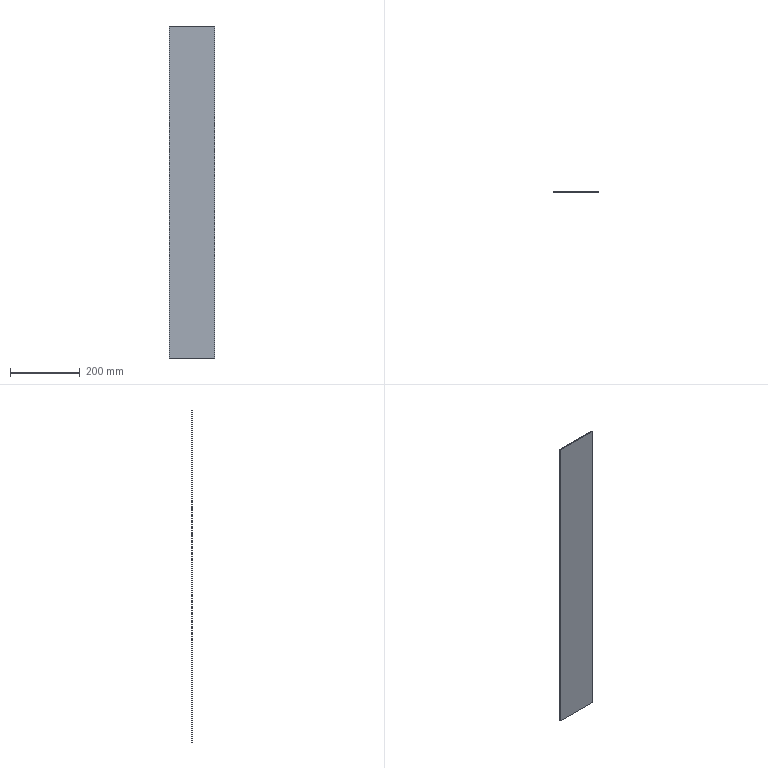Component | SolidWorks | SYM0671-81-101-1_SYM0590-81-104-2 | 1 solid | 6 faces | box 130 x 2 x 950 mm | volume 247000 mm3 | plane 6 | material Plain Carbon Steel
build123d program:
from build123d import *

# Parameters (mm, degrees)
SKETCH1_W      = 130
SKETCH1_H      = 950
EXTRUDE1_DEPTH = 2


with BuildPart() as part:
    # Sketch1 → Extrude1 (new body)
    with BuildSketch(Plane(origin=(0, 0, 0), x_dir=(1, 0, 0), z_dir=(0, 1, 0))):
        with Locations((33.603, -431.608)):
            Rectangle(SKETCH1_W, SKETCH1_H)
    extrude(amount=EXTRUDE1_DEPTH)


solid = part.part

# Placed as in the assembly
solid = solid.moved(Location((408.649, -478.857, 83.909), (0, 0, 0)))
STEP:
#1=CARTESIAN_POINT('',(14.852,-18.853,1.595));
#2=VERTEX_POINT('',#1);
#3=CARTESIAN_POINT('',(14.852,-18.853,38.997));
#4=VERTEX_POINT('',#3);
#5=CARTESIAN_POINT('',(14.852,-18.853,1.595));
#6=DIRECTION('',(0.,0.,1.));
#7=VECTOR('',#6,39.37);
#8=LINE('',#5,#7);
#9=EDGE_CURVE('',#2,#4,#8,.T.);
#10=ORIENTED_EDGE('',*,*,#9,.T.);
#11=CARTESIAN_POINT('',(14.852,-18.774,38.997));
#12=VERTEX_POINT('',#11);
#13=CARTESIAN_POINT('',(14.852,-18.774,38.997));
#14=DIRECTION('',(0.,-1.,0.));
#15=VECTOR('',#14,39.37);
#16=LINE('',#13,#15);
#17=EDGE_CURVE('',#12,#4,#16,.T.);
#18=ORIENTED_EDGE('',*,*,#17,.F.);
#19=CARTESIAN_POINT('',(14.852,-18.774,1.595));
#20=VERTEX_POINT('',#19);
#21=CARTESIAN_POINT('',(14.852,-18.774,1.595));
#22=DIRECTION('',(0.,0.,1.));
#23=VECTOR('',#22,39.37);
#24=LINE('',#21,#23);
#25=EDGE_CURVE('',#20,#12,#24,.T.);
#26=ORIENTED_EDGE('',*,*,#25,.F.);
#27=CARTESIAN_POINT('',(14.852,-18.774,1.595));
#28=DIRECTION('',(0.,-1.,0.));
#29=VECTOR('',#28,39.37);
#30=LINE('',#27,#29);
#31=EDGE_CURVE('',#20,#2,#30,.T.);
#32=ORIENTED_EDGE('',*,*,#31,.T.);
#33=EDGE_LOOP('',(#10,#18,#26,#32));
#34=FACE_OUTER_BOUND('',#33,.T.);
#35=CARTESIAN_POINT('',(14.852,-18.774,1.595));
#36=DIRECTION('',(1.,0.,-0.));
#37=DIRECTION('',(-0.,0.,-1.));
#38=AXIS2_PLACEMENT_3D('',#35,#36,#37);
#39=PLANE('',#38);
#40=ADVANCED_FACE('',(#34),#39,.F.);
#41=CARTESIAN_POINT('',(19.971,-18.853,38.997));
#42=VERTEX_POINT('',#41);
#43=CARTESIAN_POINT('',(14.852,-18.853,38.997));
#44=DIRECTION('',(1.,0.,0.));
#45=VECTOR('',#44,39.37);
#46=LINE('',#43,#45);
#47=EDGE_CURVE('',#4,#42,#46,.T.);
#48=ORIENTED_EDGE('',*,*,#47,.T.);
#49=CARTESIAN_POINT('',(19.971,-18.774,38.997));
#50=VERTEX_POINT('',#49);
#51=CARTESIAN_POINT('',(19.971,-18.774,38.997));
#52=DIRECTION('',(0.,-1.,0.));
#53=VECTOR('',#52,39.37);
#54=LINE('',#51,#53);
#55=EDGE_CURVE('',#50,#42,#54,.T.);
#56=ORIENTED_EDGE('',*,*,#55,.F.);
#57=CARTESIAN_POINT('',(14.852,-18.774,38.997));
#58=DIRECTION('',(1.,0.,0.));
#59=VECTOR('',#58,39.37);
#60=LINE('',#57,#59);
#61=EDGE_CURVE('',#12,#50,#60,.T.);
#62=ORIENTED_EDGE('',*,*,#61,.F.);
#63=ORIENTED_EDGE('',*,*,#17,.T.);
#64=EDGE_LOOP('',(#48,#56,#62,#63));
#65=FACE_OUTER_BOUND('',#64,.T.);
#66=CARTESIAN_POINT('',(14.852,-18.774,38.997));
#67=DIRECTION('',(0.,0.,-1.));
#68=DIRECTION('',(-1.,0.,0.));
#69=AXIS2_PLACEMENT_3D('',#66,#67,#68);
#70=PLANE('',#69);
#71=ADVANCED_FACE('',(#65),#70,.F.);
#72=CARTESIAN_POINT('',(19.971,-18.853,1.595));
#73=VERTEX_POINT('',#72);
#74=CARTESIAN_POINT('',(19.971,-18.853,1.595));
#75=DIRECTION('',(-0.,0.,-1.));
#76=VECTOR('',#75,39.37);
#77=LINE('',#74,#76);
#78=EDGE_CURVE('',#42,#73,#77,.T.);
#79=ORIENTED_EDGE('',*,*,#78,.T.);
#80=CARTESIAN_POINT('',(19.971,-18.774,1.595));
#81=VERTEX_POINT('',#80);
#82=CARTESIAN_POINT('',(19.971,-18.774,1.595));
#83=DIRECTION('',(0.,-1.,0.));
#84=VECTOR('',#83,39.37);
#85=LINE('',#82,#84);
#86=EDGE_CURVE('',#81,#73,#85,.T.);
#87=ORIENTED_EDGE('',*,*,#86,.F.);
#88=CARTESIAN_POINT('',(19.971,-18.774,1.595));
#89=DIRECTION('',(-0.,0.,-1.));
#90=VECTOR('',#89,39.37);
#91=LINE('',#88,#90);
#92=EDGE_CURVE('',#50,#81,#91,.T.);
#93=ORIENTED_EDGE('',*,*,#92,.F.);
#94=ORIENTED_EDGE('',*,*,#55,.T.);
#95=EDGE_LOOP('',(#79,#87,#93,#94));
#96=FACE_OUTER_BOUND('',#95,.T.);
#97=CARTESIAN_POINT('',(19.971,-18.774,1.595));
#98=DIRECTION('',(-1.,0.,0.));
#99=DIRECTION('',(0.,0.,1.));
#100=AXIS2_PLACEMENT_3D('',#97,#98,#99);
#101=PLANE('',#100);
#102=ADVANCED_FACE('',(#96),#101,.F.);
#103=CARTESIAN_POINT('',(14.852,-18.853,1.595));
#104=DIRECTION('',(-1.,0.,0.));
#105=VECTOR('',#104,39.37);
#106=LINE('',#103,#105);
#107=EDGE_CURVE('',#73,#2,#106,.T.);
#108=ORIENTED_EDGE('',*,*,#107,.T.);
#109=ORIENTED_EDGE('',*,*,#31,.F.);
#110=CARTESIAN_POINT('',(14.852,-18.774,1.595));
#111=DIRECTION('',(-1.,0.,0.));
#112=VECTOR('',#111,39.37);
#113=LINE('',#110,#112);
#114=EDGE_CURVE('',#81,#20,#113,.T.);
#115=ORIENTED_EDGE('',*,*,#114,.F.);
#116=ORIENTED_EDGE('',*,*,#86,.T.);
#117=EDGE_LOOP('',(#108,#109,#115,#116));
#118=FACE_OUTER_BOUND('',#117,.T.);
#119=CARTESIAN_POINT('',(14.852,-18.774,1.595));
#120=DIRECTION('',(0.,0.,1.));
#121=DIRECTION('',(1.,0.,0.));
#122=AXIS2_PLACEMENT_3D('',#119,#120,#121);
#123=PLANE('',#122);
#124=ADVANCED_FACE('',(#118),#123,.F.);
#125=ORIENTED_EDGE('',*,*,#25,.T.);
#126=ORIENTED_EDGE('',*,*,#61,.T.);
#127=ORIENTED_EDGE('',*,*,#92,.T.);
#128=ORIENTED_EDGE('',*,*,#114,.T.);
#129=EDGE_LOOP('',(#125,#126,#127,#128));
#130=FACE_OUTER_BOUND('',#129,.T.);
#131=CARTESIAN_POINT('',(14.852,-18.774,38.997));
#132=DIRECTION('',(0.,1.,0.));
#133=DIRECTION('',(0.,0.,1.));
#134=AXIS2_PLACEMENT_3D('',#131,#132,#133);
#135=PLANE('',#134);
#136=ADVANCED_FACE('',(#130),#135,.T.);
#137=ORIENTED_EDGE('',*,*,#9,.F.);
#138=ORIENTED_EDGE('',*,*,#107,.F.);
#139=ORIENTED_EDGE('',*,*,#78,.F.);
#140=ORIENTED_EDGE('',*,*,#47,.F.);
#141=EDGE_LOOP('',(#137,#138,#139,#140));
#142=FACE_OUTER_BOUND('',#141,.T.);
#143=CARTESIAN_POINT('',(14.852,-18.853,38.997));
#144=DIRECTION('',(0.,1.,0.));
#145=DIRECTION('',(0.,0.,1.));
#146=AXIS2_PLACEMENT_3D('',#143,#144,#145);
#147=PLANE('',#146);
#148=ADVANCED_FACE('',(#142),#147,.F.);
#149=CLOSED_SHELL('',(#40,#71,#102,#124,#136,#148));
#150=MANIFOLD_SOLID_BREP('',#149);
#151=CARTESIAN_POINT('',(0.,0.,0.));
#152=DIRECTION('',(0.,0.,1.));
#153=DIRECTION('',(1.,0.,0.));
#154=AXIS2_PLACEMENT_3D('',#151,#152,#153);
#155=(LENGTH_UNIT()NAMED_UNIT(*)SI_UNIT($,.METRE.));
#156=LENGTH_MEASURE_WITH_UNIT(LENGTH_MEASURE(0.0254),#155);
#157=DIMENSIONAL_EXPONENTS(1.,0.,0.,0.,0.,0.,0.);
#158=(CONVERSION_BASED_UNIT('',#156)LENGTH_UNIT()NAMED_UNIT(#157));
#159=UNCERTAINTY_MEASURE_WITH_UNIT(LENGTH_MEASURE(0.00001),#158,'','');
#160=(NAMED_UNIT(*)PLANE_ANGLE_UNIT()SI_UNIT($,.RADIAN.));
#161=(NAMED_UNIT(*)SI_UNIT($,.STERADIAN.)SOLID_ANGLE_UNIT());
#162=(GEOMETRIC_REPRESENTATION_CONTEXT(3)GLOBAL_UNCERTAINTY_ASSIGNED_CONTEXT((#159))GLOBAL_UNIT_ASSIGNED_CONTEXT((#158,#160,#161))REPRESENTATION_CONTEXT('',''));
#163=ADVANCED_BREP_SHAPE_REPRESENTATION('',(#150,#154),#162);
#164=COLOUR_RGB('',0.7922,0.8196,0.9333);
#165=FILL_AREA_STYLE_COLOUR('',#164);
#166=FILL_AREA_STYLE('',(#165));
#167=SURFACE_STYLE_FILL_AREA(#166);
#168=SURFACE_SIDE_STYLE('',(#167));
#169=SURFACE_STYLE_USAGE(.BOTH.,#168);
#170=PRESENTATION_STYLE_ASSIGNMENT((#169));
#171=STYLED_ITEM('',(#170),#150);
#172=PRESENTATION_LAYER_ASSIGNMENT('','',(#171));
#173=(LENGTH_UNIT()NAMED_UNIT(*)SI_UNIT($,.METRE.));
#174=LENGTH_MEASURE_WITH_UNIT(LENGTH_MEASURE(0.0254),#173);
#175=DIMENSIONAL_EXPONENTS(1.,0.,0.,0.,0.,0.,0.);
#176=(CONVERSION_BASED_UNIT('',#174)LENGTH_UNIT()NAMED_UNIT(#175));
#177=UNCERTAINTY_MEASURE_WITH_UNIT(LENGTH_MEASURE(0.00001),#176,'','');
#178=(NAMED_UNIT(*)PLANE_ANGLE_UNIT()SI_UNIT($,.RADIAN.));
#179=(NAMED_UNIT(*)SI_UNIT($,.STERADIAN.)SOLID_ANGLE_UNIT());
#180=(GEOMETRIC_REPRESENTATION_CONTEXT(3)GLOBAL_UNCERTAINTY_ASSIGNED_CONTEXT((#177))GLOBAL_UNIT_ASSIGNED_CONTEXT((#176,#178,#179))REPRESENTATION_CONTEXT('',''));
#181=MECHANICAL_DESIGN_GEOMETRIC_PRESENTATION_REPRESENTATION('',(#171),#180);